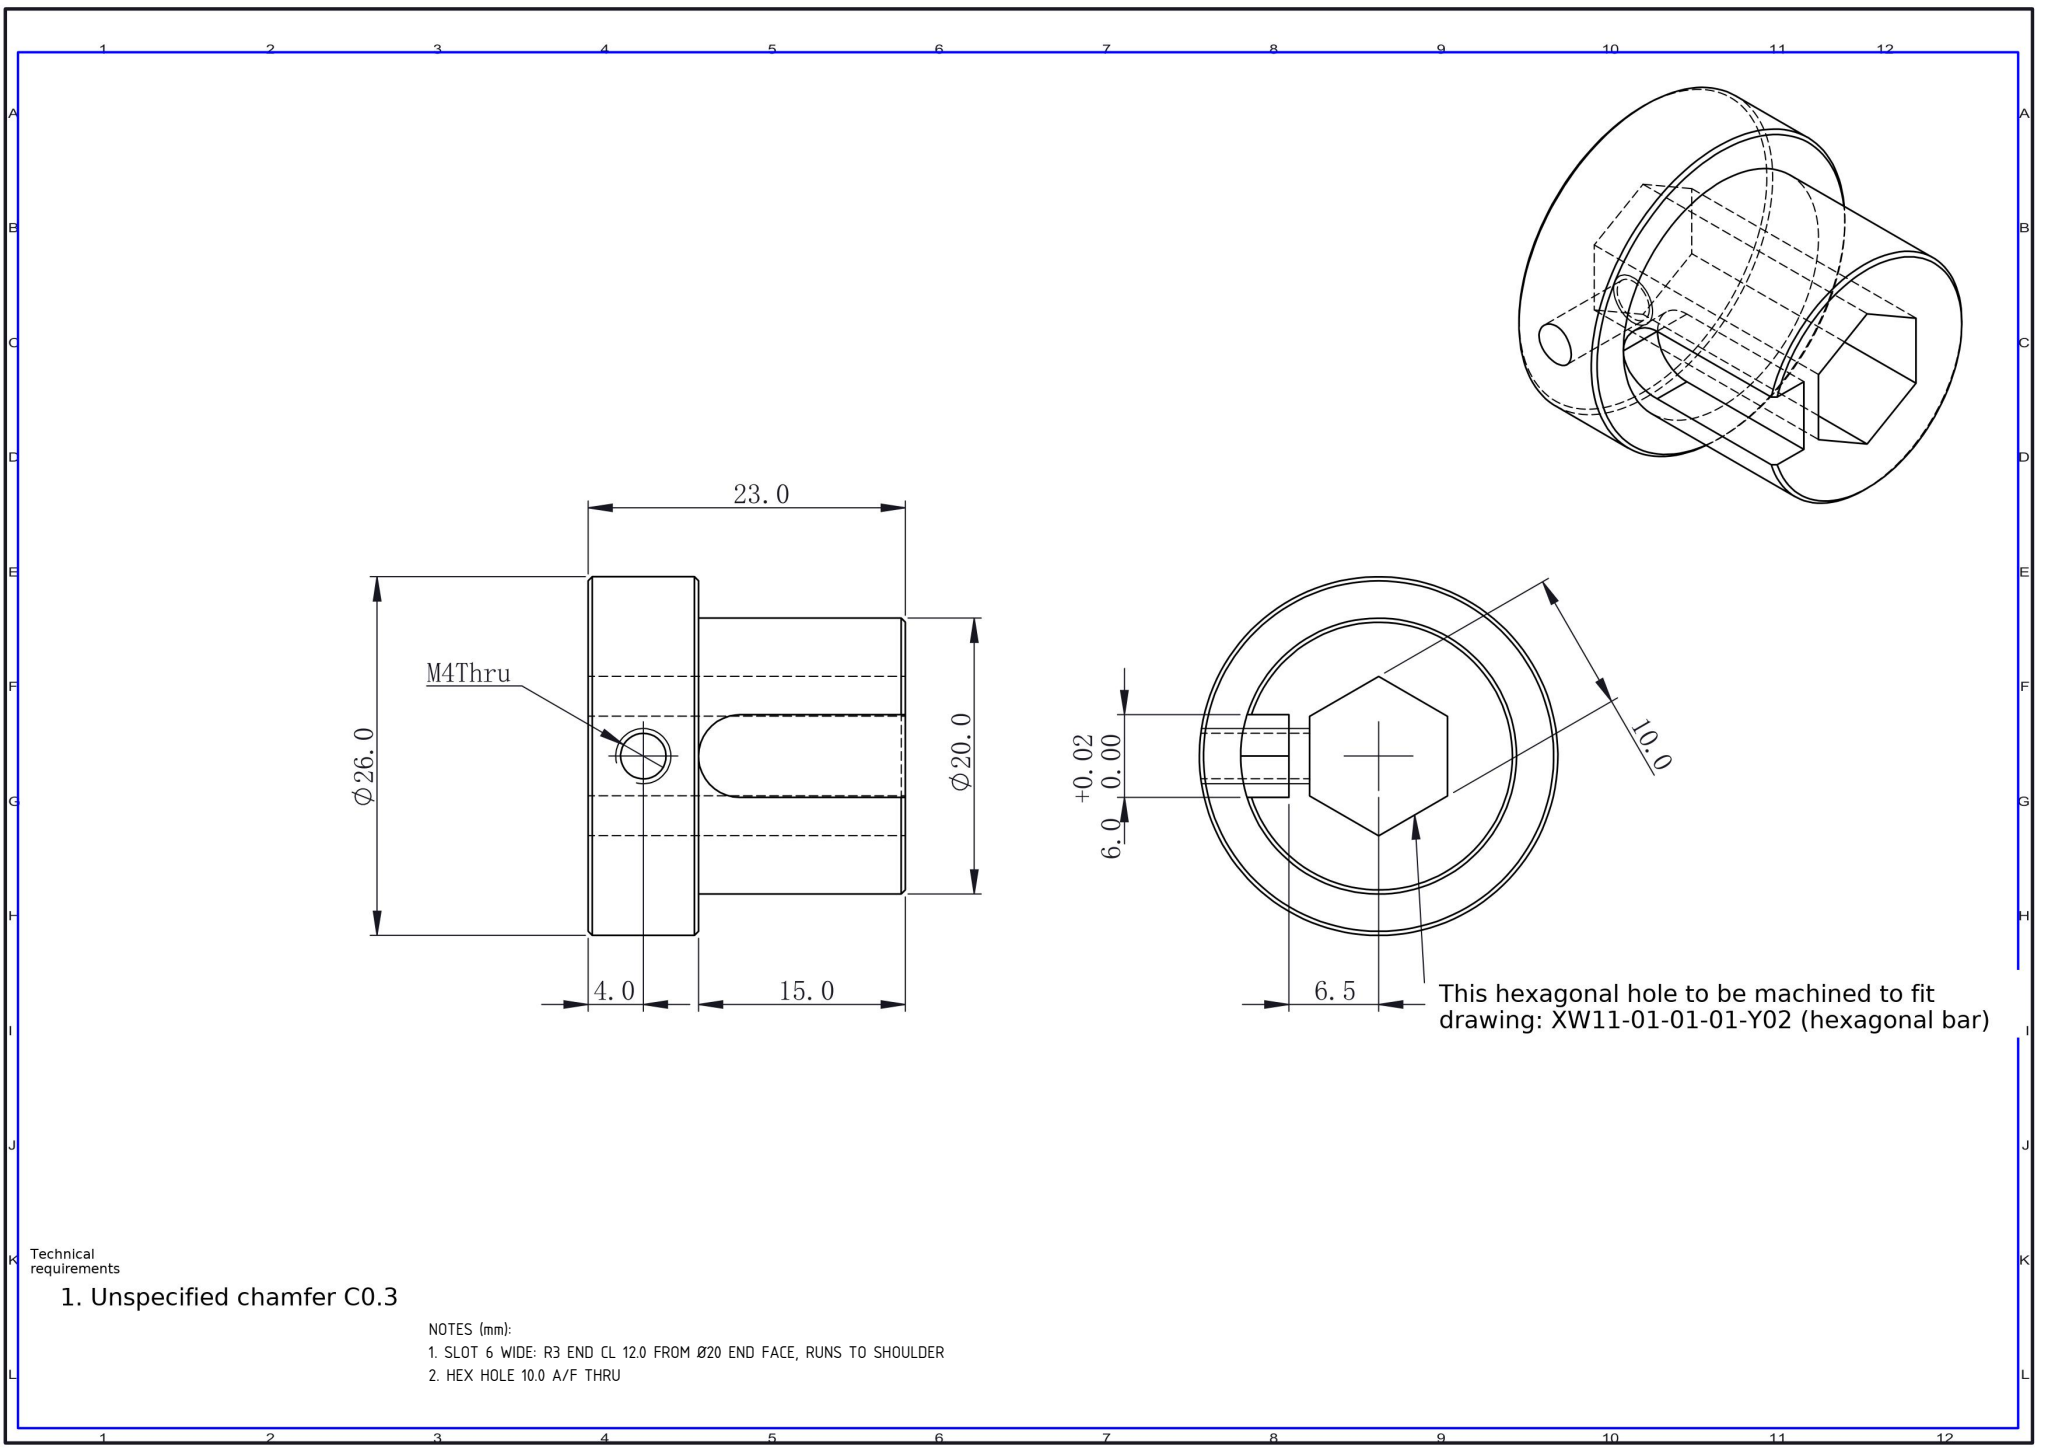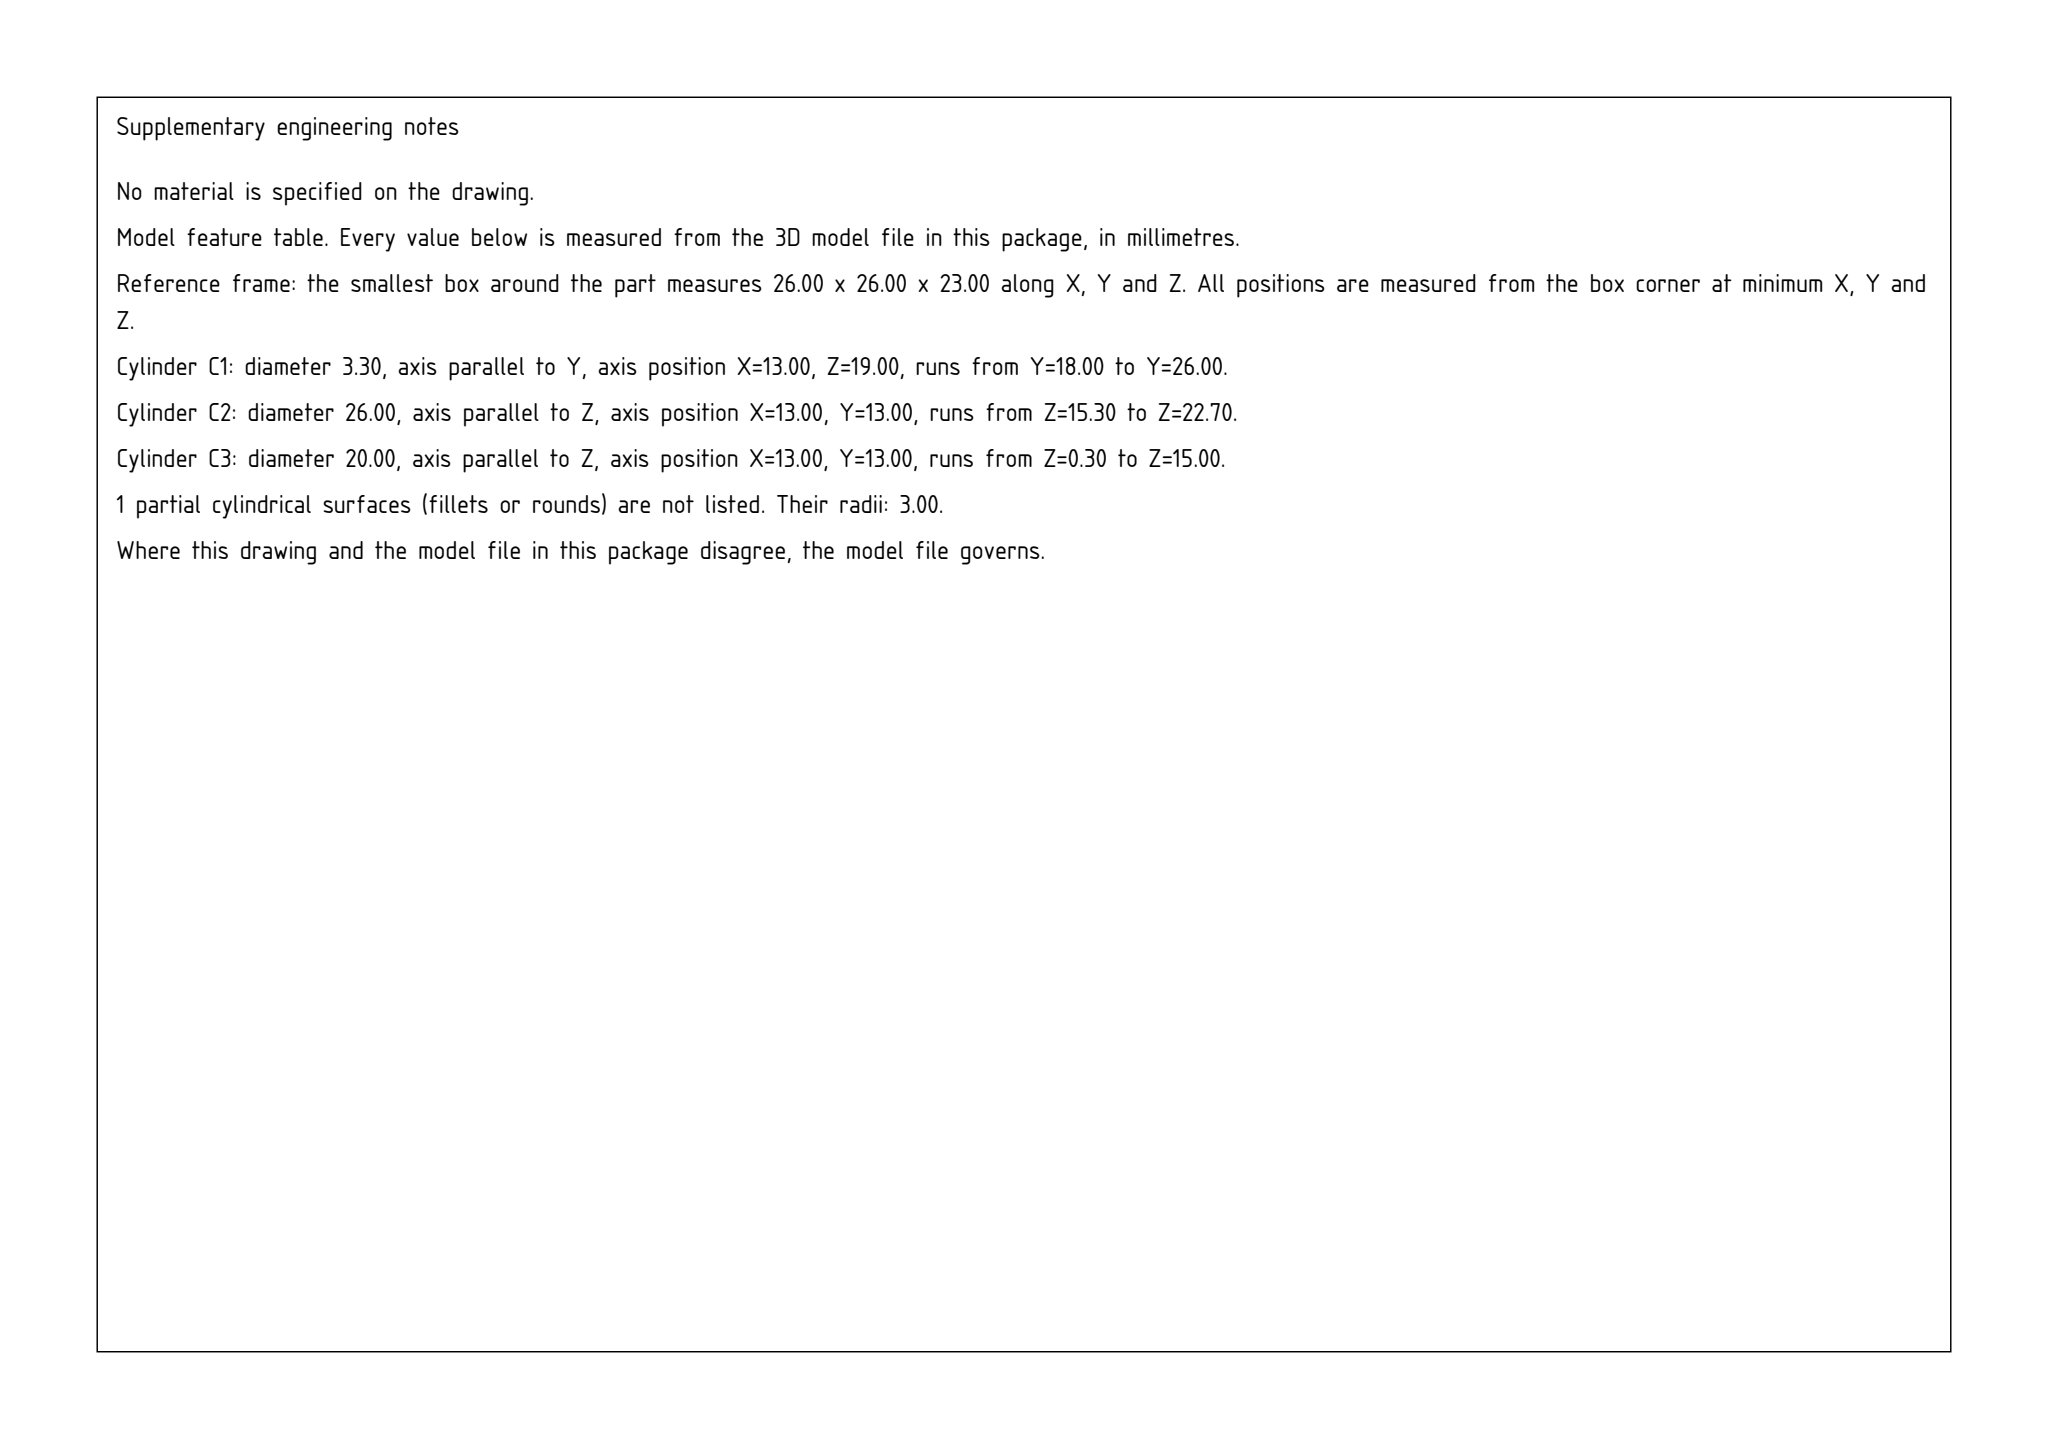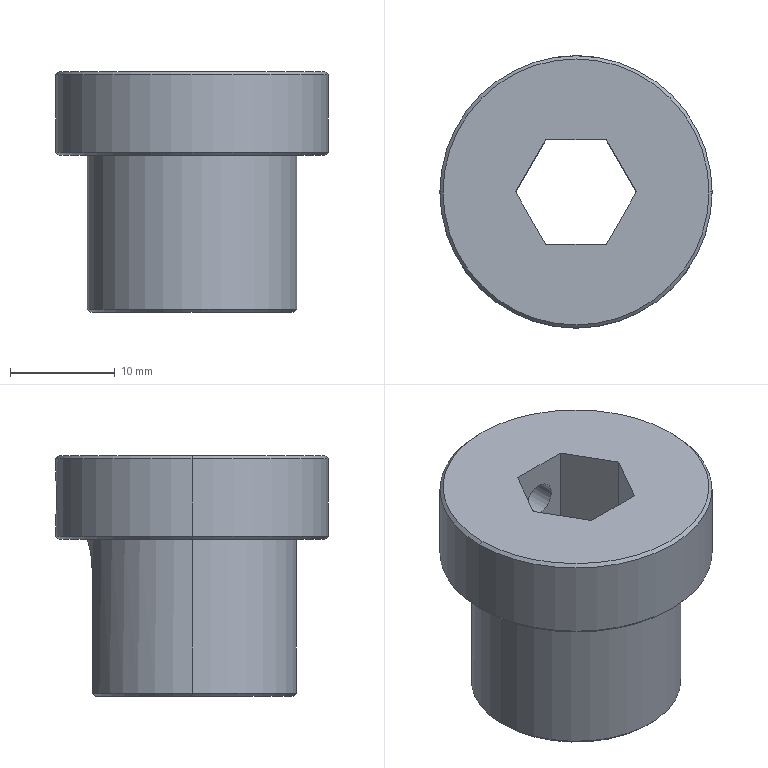Part | SolidWorks | mm | 1 solid | 28 faces | box 26 x 26 x 23 mm | volume 6601 mm3 | plane 12 | cylinder 9 | cone 7 | commonest cylinder face diameters 20 x3 3.3 x2 26 x2 6 x2
Drawing notes:
SLOT 6 WIDE: R3 END CL 12.0 FROM Ø20 END FACE, RUNS TO SHOULDER | from the solid: cyl dia 6.0 axis y at z=12.0 (x=13.0), len 3.5; shoulder plane z=15.0; Ø20 end face z=0; slot width 6.0, depth to x=16.0 (6.5 from Ø26 OD side per 6.5 dim)
HEX HOLE 10.0 A/F THRU | from the solid: Hex flats are planes y=8 and y=18 (10.0 across flats); only z-planes are 0, 15 (shoulder) and 23 (flange face), so no pocket bottom exists; M4 Ø3.3 hole at z=19 is split into two 8.0 lengths (y 0-8, 18-26) by the hex, proving it runs through the full 23.0 length.